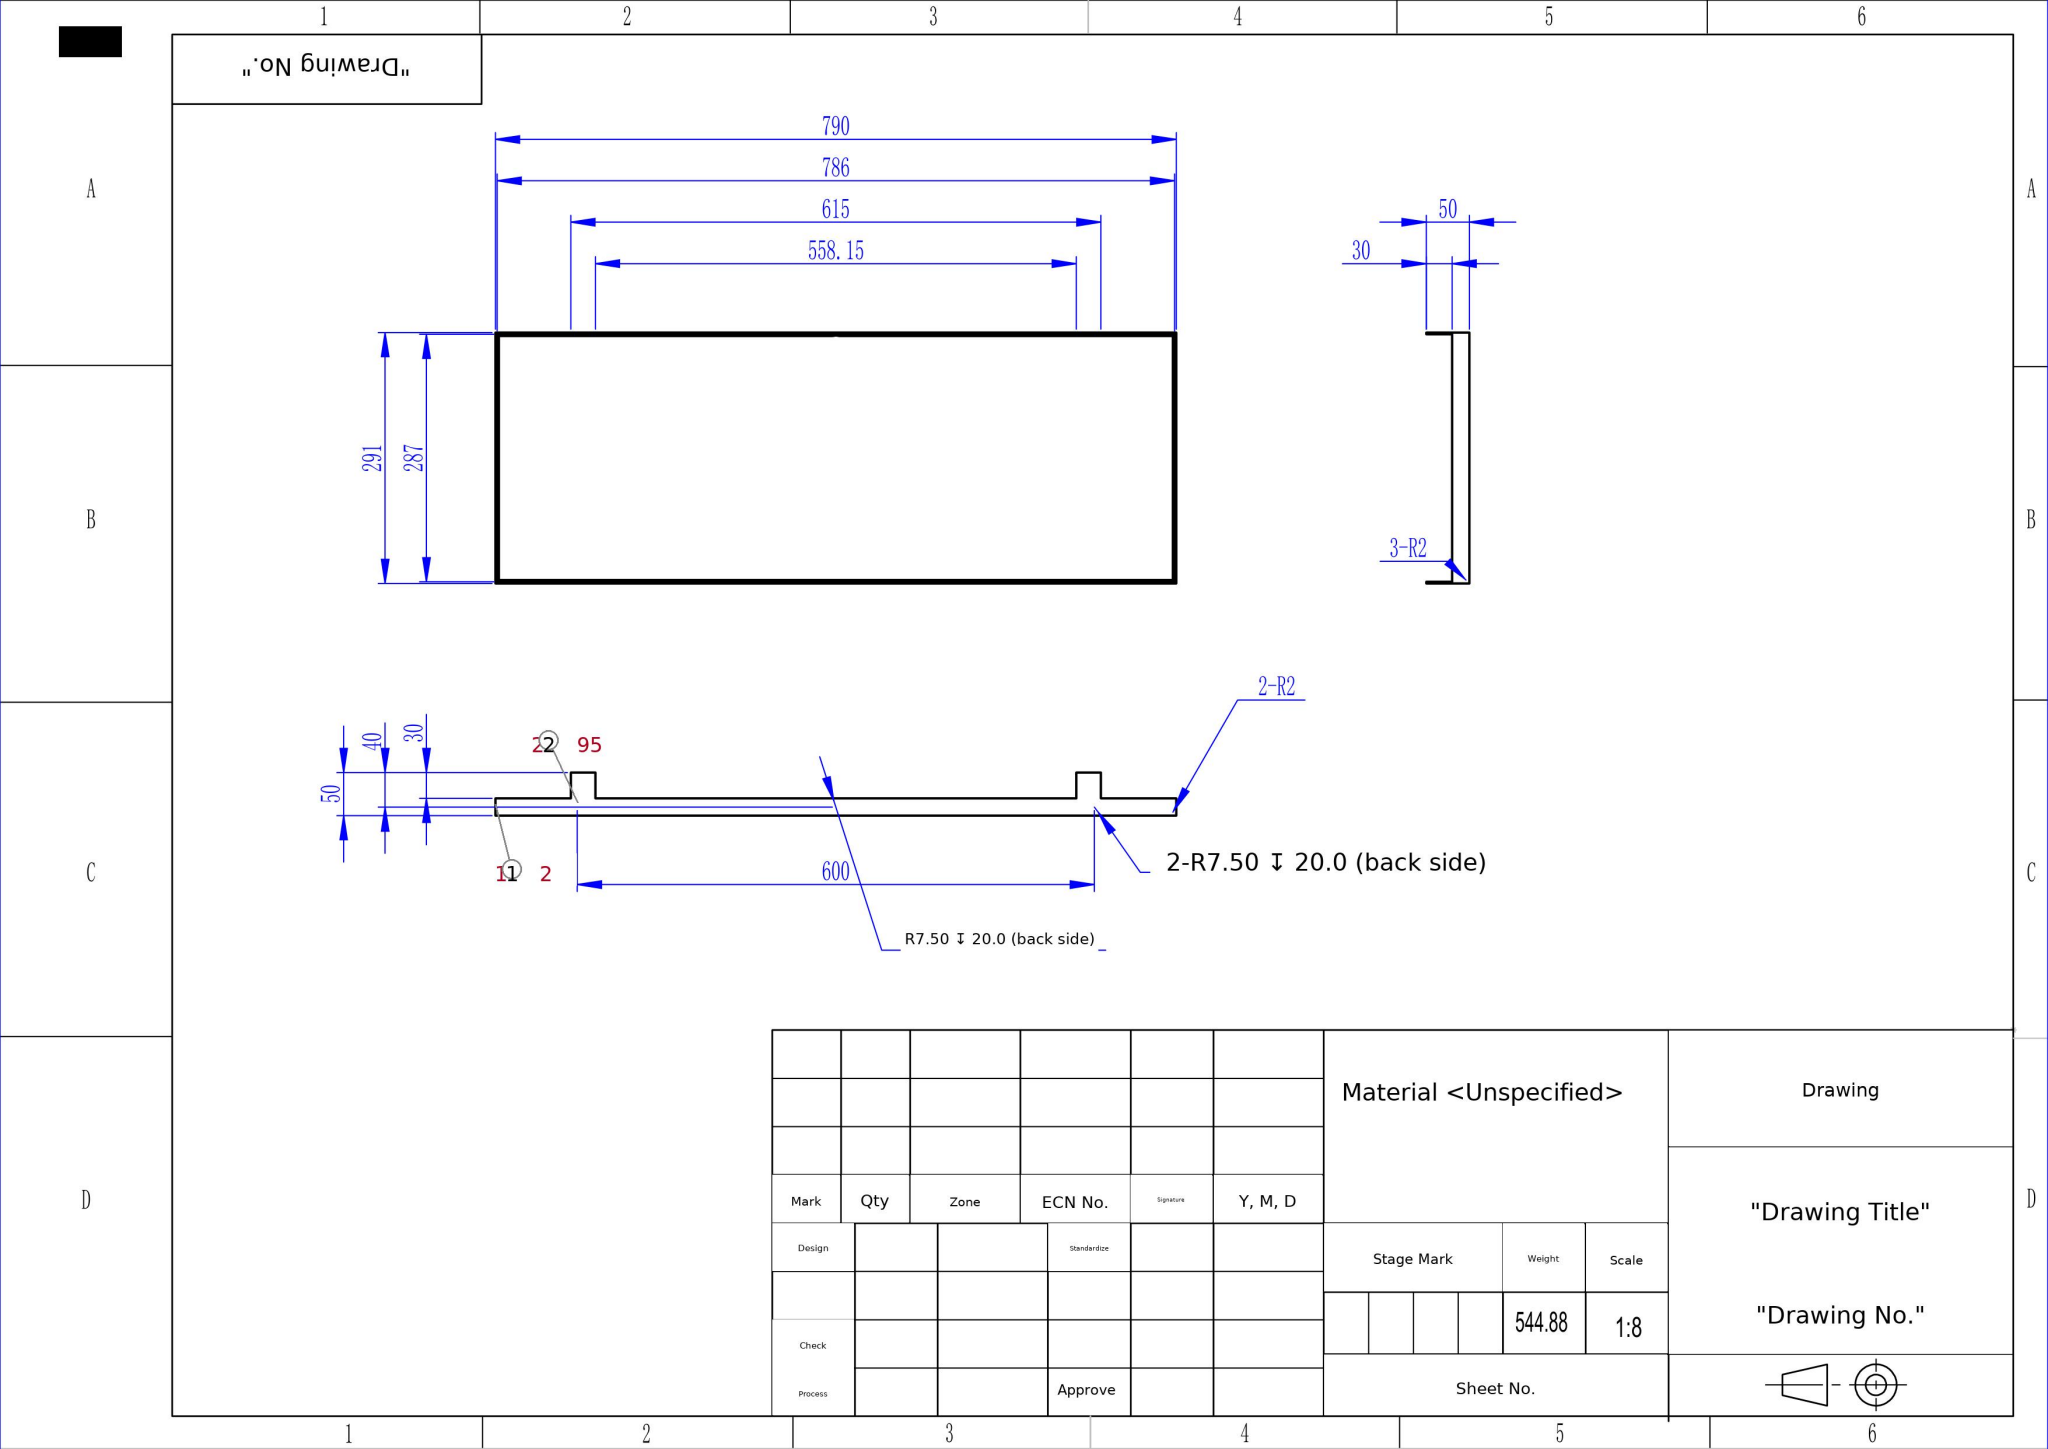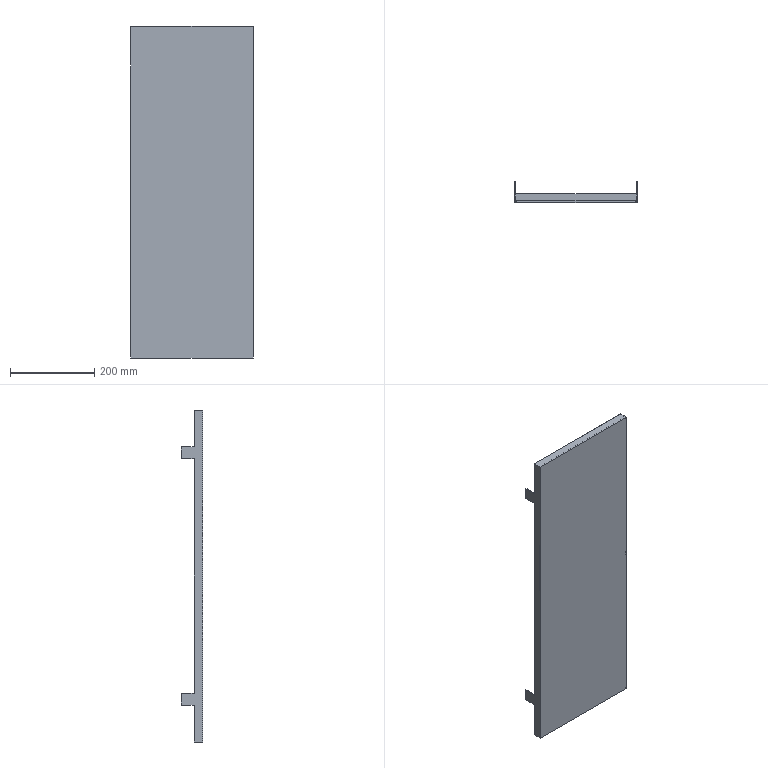Part | SolidWorks | mm | 1 solid | 38 faces | box 291 x 50 x 790 mm | volume 544919 mm3 | plane 26 | cylinder 11 | spline 1 | commonest cylinder face diameters 15 x6 4 x5